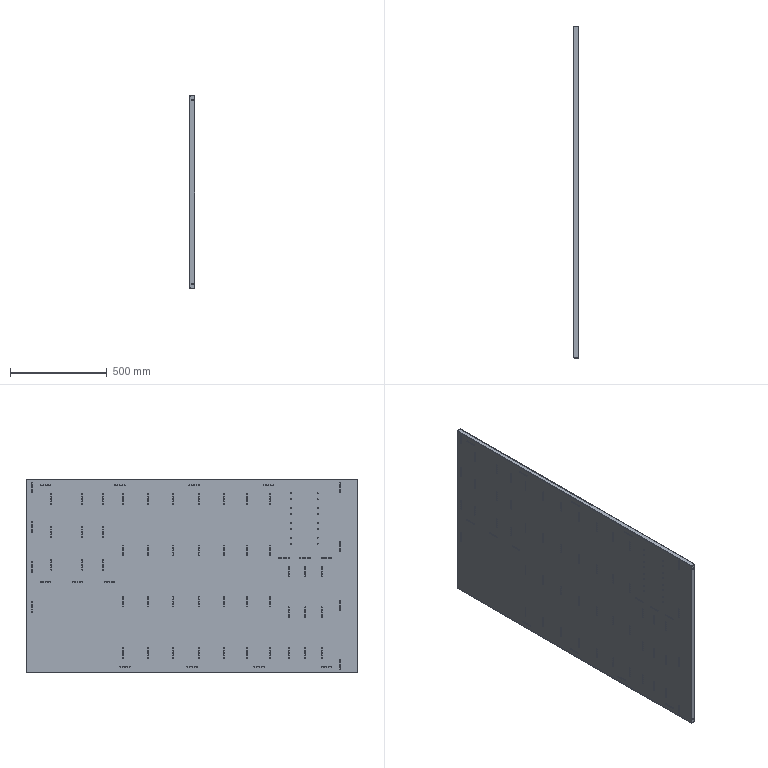Component | SolidWorks | Shelf-1 | 1 solid | 830 faces | volume 3493909 mm3 | cylinder 764 | plane 54 | spline 12 | commonest cylinder face diameters 5 x712 4 x24 8 x8 0.2 x8 3.8 x8 7.99 x4